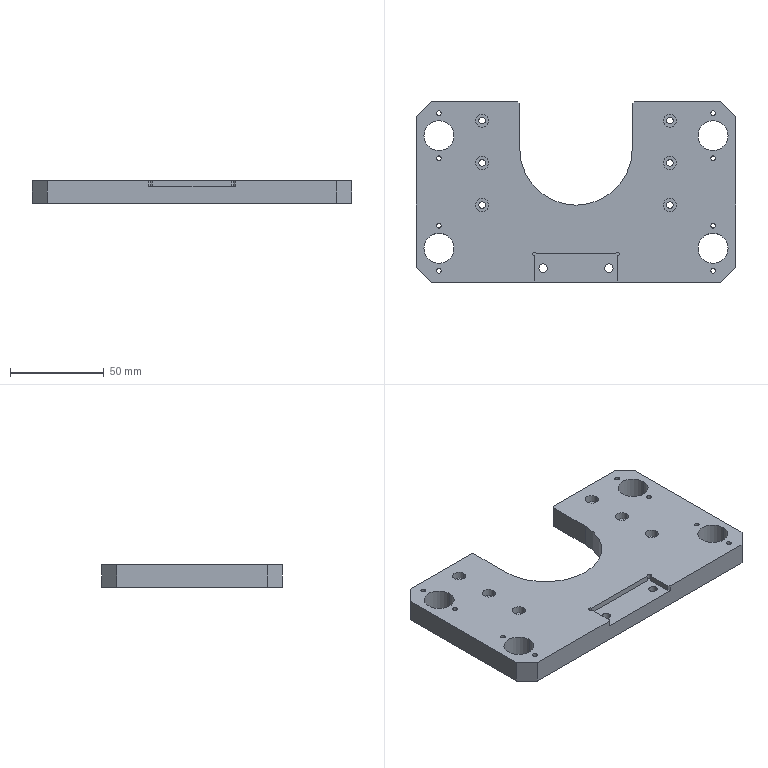Component | SolidWorks | 170423A4-SafetyPowerProbeFixingPlate3-1 | 1 solid | 107 faces | box 170 x 96 x 12 mm | volume 142565 mm3 | cylinder 66 | plane 41 | commonest cylinder face diameters 2.5 x16 7 x12 3.5 x12 2 x9 16 x8 9 x4 4.5 x4 60 x1
build123d program:
from build123d import *

# Parameters (mm, degrees)
SKETCH1_W                                       = 170
SKETCH1_H                                       = 96
BOSS_EXTRUDE1_DEPTH                             = 12
SKETCH2_W                                       = 10.1
SKETCH2_H                                       = 65
CUT_EXTRUDE1_DEPTH                              = 2
CUT_EXTRUDE4_DEPTH                              = 99.127
CUT_EXTRUDE4_DEPTH_BACK                         = 99.127
SKETCH7_R                                       = 8
SKETCH8_W                                       = 44.2
SKETCH8_H                                       = 15
CUT_EXTRUDE5_DEPTH                              = 3
CHAMFER1_SIZE                                   = 8
SKETCH9_R                                       = 1
CUT_EXTRUDE6_DEPTH                              = 2
M4_HEX_SOCKET_HEAD_CAP_SCREW_CBORE1_D           = 4.5
M4_HEX_SOCKET_HEAD_CAP_SCREW_CBORE1_CBORE_D     = 9
M4_HEX_SOCKET_HEAD_CAP_SCREW_CBORE1_CBORE_DEPTH = 4.5
M3_HEX_SOCKET_HEAD_CAP_SCREW_CBORE1_D           = 3.5
M3_HEX_SOCKET_HEAD_CAP_SCREW_CBORE1_CBORE_D     = 7
M3_HEX_SOCKET_HEAD_CAP_SCREW_CBORE1_CBORE_DEPTH = 4
SKETCH16_R                                      = 1
CUT_EXTRUDE7_DEPTH                              = 3
M3_TAPPED_HOLE1_D                               = 2.5
CUT_EXTRUDE8_DEPTH                              = 99.351
CHAMFER2_SIZE                                   = 1


with BuildPart() as part:
    # Sketch1 → Boss-Extrude1 (new body)
    with BuildSketch(Plane.XY):
        Rectangle(SKETCH1_W, SKETCH1_H)
    extrude(amount=BOSS_EXTRUDE1_DEPTH)

    # Sketch2 → Cut-Extrude1 (cut)
    with BuildSketch(Plane.XY.offset(12)):
        with Locations((-50, -15.5)):
            Rectangle(SKETCH2_W, SKETCH2_H)
        with Locations((50, -15.5)):
            Rectangle(SKETCH2_W, SKETCH2_H)
    extrude(amount=-CUT_EXTRUDE1_DEPTH, mode=Mode.SUBTRACT)

    # Sketch7 → Cut-Extrude4 (cut, two sides: drawn at the far end of the back side and taken through both)
    with BuildSketch(Plane.XY.offset(10).offset(-CUT_EXTRUDE4_DEPTH_BACK)):
        with Locations((-73, 30)):
            Circle(SKETCH7_R)
        with Locations((-73, -30)):
            Circle(SKETCH7_R)
        with Locations((73, 30)):
            Circle(SKETCH7_R)
        with Locations((73, -30)):
            Circle(SKETCH7_R)
    extrude(amount=CUT_EXTRUDE4_DEPTH + CUT_EXTRUDE4_DEPTH_BACK, mode=Mode.SUBTRACT)

    # Sketch8 → Cut-Extrude5 (cut)
    with BuildSketch(Plane.XY):
        with Locations((0, 40.5)):
            Rectangle(SKETCH8_W, SKETCH8_H)
    extrude(amount=CUT_EXTRUDE5_DEPTH, mode=Mode.SUBTRACT)

    # Chamfer1
    chamfer1_edges = [part.edges().sort_by_distance(p)[0] for p in [
        (85, -48, 6),
        (-85, -48, 6),
        (-85, 48, 6),
        (85, 48, 6),
    ]]
    chamfer(chamfer1_edges, length=CHAMFER1_SIZE)

    # Sketch9 → Cut-Extrude6 (cut)
    with BuildSketch(Plane.XY.offset(12)):
        with Locations((-55.05, 17)):
            Circle(SKETCH9_R)
        with Locations((-44.95, 17)):
            Circle(SKETCH9_R)
        with Locations((44.95, 17)):
            Circle(SKETCH9_R)
        with Locations((55.05, 17)):
            Circle(SKETCH9_R)
    extrude(amount=-CUT_EXTRUDE6_DEPTH, mode=Mode.SUBTRACT)

    # M4 Hex Socket Head Cap Screw CBORE1 (through all)
    with Locations(Plane.XY.offset(12)):
        with Locations((17.5, 40.5), (-17.5, 40.5)):
            CounterBoreHole(M4_HEX_SOCKET_HEAD_CAP_SCREW_CBORE1_D / 2, M4_HEX_SOCKET_HEAD_CAP_SCREW_CBORE1_CBORE_D / 2, M4_HEX_SOCKET_HEAD_CAP_SCREW_CBORE1_CBORE_DEPTH)

    # M3 Hex Socket Head Cap Screw CBORE1 (through all)
    with Locations(Plane(origin=(0, 0, 0), x_dir=(-1, 0, 0), z_dir=(0, 0, -1))):
        with Locations((50, -38), (50, -15.5), (50, 7), (-50, 7), (-50, -15.5), (-50, -38)):
            CounterBoreHole(M3_HEX_SOCKET_HEAD_CAP_SCREW_CBORE1_D / 2, M3_HEX_SOCKET_HEAD_CAP_SCREW_CBORE1_CBORE_D / 2, M3_HEX_SOCKET_HEAD_CAP_SCREW_CBORE1_CBORE_DEPTH)

    # Sketch16 → Cut-Extrude7 (cut)
    with BuildSketch(Plane(origin=(0, 0, 0), x_dir=(-1, 0, 0), z_dir=(0, 0, -1))):
        with Locations((-22.1, 33)):
            Circle(SKETCH16_R)
        with Locations((22.1, 33)):
            Circle(SKETCH16_R)
    extrude(amount=-CUT_EXTRUDE7_DEPTH, mode=Mode.SUBTRACT)

    # M3 Tapped Hole1 (through all)
    with Locations(Plane.XY.offset(12)):
        with Locations((-73, 42), (-73, 18), (-73, -18), (-73, -42), (73, -42), (73, -18), (73, 18), (73, 42)):
            Hole(M3_TAPPED_HOLE1_D / 2)

    # Sketch19 → Cut-Extrude8 (cut, through all)
    with BuildSketch(Plane.XY.offset(12)):
        with BuildLine():
            Line((-30, -48), (-30, -23))
            ThreePointArc((-30, -23), (0, 7), (30, -23))
            Line((30, -23), (30, -48))
            ThreePointArc((30, -48), (0, -78), (-30, -48))
        make_face()
    extrude(amount=-CUT_EXTRUDE8_DEPTH, mode=Mode.SUBTRACT)

    # Chamfer2
    chamfer2_edges = [part.edges().sort_by_distance(p)[0] for p in [
        (-55.05, -48, 11),
        (-44.95, -48, 11),
        (30, -48, 6),
        (-30, -48, 6),
        (55.05, -48, 11),
        (44.95, -48, 11),
        (22.1, 48, 1.5),
        (-22.1, 48, 1.5),
    ]]
    chamfer(chamfer2_edges, length=CHAMFER2_SIZE)


solid = part.part

# Placed as in the assembly
solid = solid.moved(Location((28.687, -8.611, 9.926), (180, 0, 0)))